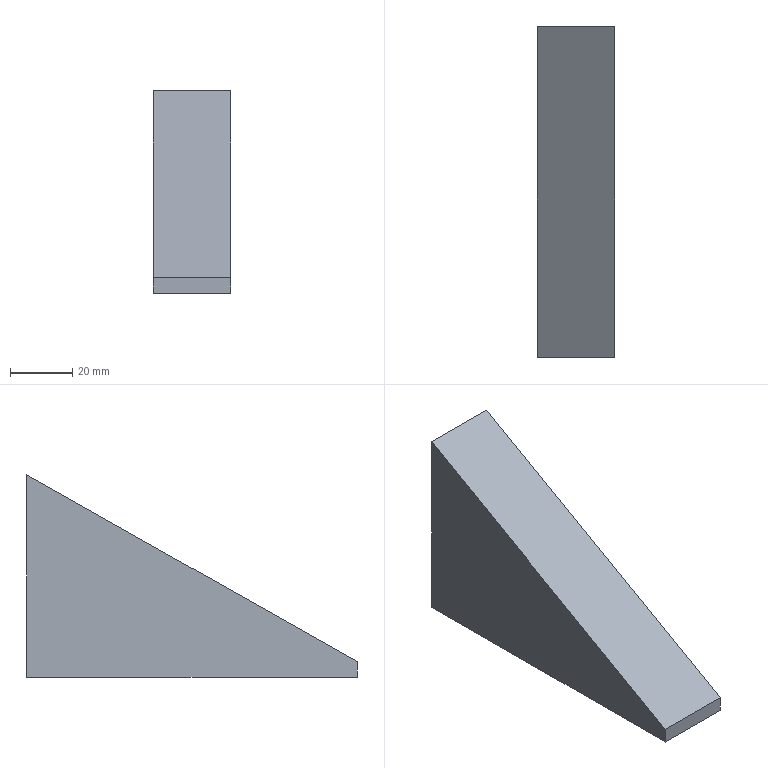Component | SolidWorks | MiddleHousing-1_Stiffener2-1 | 1 solid | 6 faces | box 25 x 106 x 65 mm | volume 92750 mm3 | plane 6
STEP:
#1=COLOUR_RGB('',0.7922,0.8196,0.9333);
#2=FILL_AREA_STYLE_COLOUR('',#1);
#3=FILL_AREA_STYLE('',(#2));
#4=SURFACE_STYLE_FILL_AREA(#3);
#5=SURFACE_SIDE_STYLE('',(#4));
#6=SURFACE_STYLE_USAGE(.BOTH.,#5);
#7=PRESENTATION_STYLE_ASSIGNMENT((#6));
#8=CARTESIAN_POINT('',(4.331,1.181,6.496));
#9=VERTEX_POINT('',#8);
#10=CARTESIAN_POINT('',(4.331,5.354,8.858));
#11=VERTEX_POINT('',#10);
#12=CARTESIAN_POINT('',(4.331,1.181,6.496));
#13=DIRECTION('',(0.,0.8703,0.4926));
#14=VECTOR('',#13,39.37);
#15=LINE('',#12,#14);
#16=EDGE_CURVE('',#9,#11,#15,.T.);
#17=ORIENTED_EDGE('',*,*,#16,.F.);
#18=CARTESIAN_POINT('',(4.331,1.181,6.299));
#19=VERTEX_POINT('',#18);
#20=CARTESIAN_POINT('',(4.331,1.181,8.858));
#21=DIRECTION('',(0.,0.,1.));
#22=VECTOR('',#21,39.37);
#23=LINE('',#20,#22);
#24=EDGE_CURVE('',#19,#9,#23,.T.);
#25=ORIENTED_EDGE('',*,*,#24,.F.);
#26=CARTESIAN_POINT('',(4.331,5.354,6.299));
#27=VERTEX_POINT('',#26);
#28=CARTESIAN_POINT('',(4.331,5.354,6.299));
#29=DIRECTION('',(0.,-1.,0.));
#30=VECTOR('',#29,39.37);
#31=LINE('',#28,#30);
#32=EDGE_CURVE('',#27,#19,#31,.T.);
#33=ORIENTED_EDGE('',*,*,#32,.F.);
#34=CARTESIAN_POINT('',(4.331,5.354,8.858));
#35=DIRECTION('',(0.,0.,-1.));
#36=VECTOR('',#35,39.37);
#37=LINE('',#34,#36);
#38=EDGE_CURVE('',#11,#27,#37,.T.);
#39=ORIENTED_EDGE('',*,*,#38,.F.);
#40=EDGE_LOOP('',(#17,#25,#33,#39));
#41=FACE_OUTER_BOUND('',#40,.T.);
#42=CARTESIAN_POINT('',(4.331,5.354,8.858));
#43=DIRECTION('',(-1.,0.,0.));
#44=DIRECTION('',(0.,0.,1.));
#45=AXIS2_PLACEMENT_3D('',#42,#43,#44);
#46=PLANE('',#45);
#47=ADVANCED_FACE('',(#41),#46,.F.);
#48=CARTESIAN_POINT('',(3.346,5.354,8.858));
#49=VERTEX_POINT('',#48);
#50=CARTESIAN_POINT('',(3.346,5.354,6.299));
#51=VERTEX_POINT('',#50);
#52=CARTESIAN_POINT('',(3.346,5.354,8.858));
#53=DIRECTION('',(0.,0.,-1.));
#54=VECTOR('',#53,39.37);
#55=LINE('',#52,#54);
#56=EDGE_CURVE('',#49,#51,#55,.T.);
#57=ORIENTED_EDGE('',*,*,#56,.F.);
#58=CARTESIAN_POINT('',(3.346,5.354,8.858));
#59=DIRECTION('',(-1.,0.,0.));
#60=VECTOR('',#59,39.37);
#61=LINE('',#58,#60);
#62=EDGE_CURVE('',#11,#49,#61,.T.);
#63=ORIENTED_EDGE('',*,*,#62,.F.);
#64=ORIENTED_EDGE('',*,*,#38,.T.);
#65=CARTESIAN_POINT('',(3.346,5.354,6.299));
#66=DIRECTION('',(1.,0.,0.));
#67=VECTOR('',#66,39.37);
#68=LINE('',#65,#67);
#69=EDGE_CURVE('',#51,#27,#68,.T.);
#70=ORIENTED_EDGE('',*,*,#69,.F.);
#71=EDGE_LOOP('',(#57,#63,#64,#70));
#72=FACE_OUTER_BOUND('',#71,.T.);
#73=CARTESIAN_POINT('',(3.346,5.354,8.858));
#74=DIRECTION('',(0.,-1.,0.));
#75=DIRECTION('',(0.,0.,-1.));
#76=AXIS2_PLACEMENT_3D('',#73,#74,#75);
#77=PLANE('',#76);
#78=ADVANCED_FACE('',(#72),#77,.F.);
#79=CARTESIAN_POINT('',(3.346,1.181,6.496));
#80=VERTEX_POINT('',#79);
#81=CARTESIAN_POINT('',(3.346,1.181,6.496));
#82=DIRECTION('',(0.,0.8703,0.4926));
#83=VECTOR('',#82,39.37);
#84=LINE('',#81,#83);
#85=EDGE_CURVE('',#80,#49,#84,.T.);
#86=ORIENTED_EDGE('',*,*,#85,.F.);
#87=CARTESIAN_POINT('',(20.276,1.181,6.496));
#88=DIRECTION('',(-1.,0.,0.));
#89=VECTOR('',#88,39.37);
#90=LINE('',#87,#89);
#91=EDGE_CURVE('',#9,#80,#90,.T.);
#92=ORIENTED_EDGE('',*,*,#91,.F.);
#93=ORIENTED_EDGE('',*,*,#16,.T.);
#94=ORIENTED_EDGE('',*,*,#62,.T.);
#95=EDGE_LOOP('',(#86,#92,#93,#94));
#96=FACE_OUTER_BOUND('',#95,.T.);
#97=CARTESIAN_POINT('',(20.276,1.181,6.496));
#98=DIRECTION('',(0.,0.4926,-0.8703));
#99=DIRECTION('',(0.,0.8703,0.4926));
#100=AXIS2_PLACEMENT_3D('',#97,#98,#99);
#101=PLANE('',#100);
#102=ADVANCED_FACE('',(#96),#101,.F.);
#103=ORIENTED_EDGE('',*,*,#91,.T.);
#104=CARTESIAN_POINT('',(3.346,1.181,6.299));
#105=VERTEX_POINT('',#104);
#106=CARTESIAN_POINT('',(3.346,1.181,8.858));
#107=DIRECTION('',(0.,0.,1.));
#108=VECTOR('',#107,39.37);
#109=LINE('',#106,#108);
#110=EDGE_CURVE('',#105,#80,#109,.T.);
#111=ORIENTED_EDGE('',*,*,#110,.F.);
#112=CARTESIAN_POINT('',(3.346,1.181,6.299));
#113=DIRECTION('',(-1.,0.,0.));
#114=VECTOR('',#113,39.37);
#115=LINE('',#112,#114);
#116=EDGE_CURVE('',#19,#105,#115,.T.);
#117=ORIENTED_EDGE('',*,*,#116,.F.);
#118=ORIENTED_EDGE('',*,*,#24,.T.);
#119=EDGE_LOOP('',(#103,#111,#117,#118));
#120=FACE_OUTER_BOUND('',#119,.T.);
#121=CARTESIAN_POINT('',(3.346,1.181,8.858));
#122=DIRECTION('',(0.,1.,0.));
#123=DIRECTION('',(0.,0.,1.));
#124=AXIS2_PLACEMENT_3D('',#121,#122,#123);
#125=PLANE('',#124);
#126=ADVANCED_FACE('',(#120),#125,.F.);
#127=ORIENTED_EDGE('',*,*,#69,.T.);
#128=ORIENTED_EDGE('',*,*,#32,.T.);
#129=ORIENTED_EDGE('',*,*,#116,.T.);
#130=CARTESIAN_POINT('',(3.346,0.9843,6.299));
#131=DIRECTION('',(0.,-1.,0.));
#132=VECTOR('',#131,39.37);
#133=LINE('',#130,#132);
#134=EDGE_CURVE('',#51,#105,#133,.T.);
#135=ORIENTED_EDGE('',*,*,#134,.F.);
#136=EDGE_LOOP('',(#127,#128,#129,#135));
#137=FACE_OUTER_BOUND('',#136,.T.);
#138=CARTESIAN_POINT('',(8.268,0.9843,6.299));
#139=DIRECTION('',(0.,0.,1.));
#140=DIRECTION('',(1.,0.,0.));
#141=AXIS2_PLACEMENT_3D('',#138,#139,#140);
#142=PLANE('',#141);
#143=ADVANCED_FACE('',(#137),#142,.F.);
#144=ORIENTED_EDGE('',*,*,#85,.T.);
#145=ORIENTED_EDGE('',*,*,#56,.T.);
#146=ORIENTED_EDGE('',*,*,#134,.T.);
#147=ORIENTED_EDGE('',*,*,#110,.T.);
#148=EDGE_LOOP('',(#144,#145,#146,#147));
#149=FACE_OUTER_BOUND('',#148,.T.);
#150=CARTESIAN_POINT('',(3.346,5.354,8.858));
#151=DIRECTION('',(1.,0.,0.));
#152=DIRECTION('',(0.,0.,-1.));
#153=AXIS2_PLACEMENT_3D('',#150,#151,#152);
#154=PLANE('',#153);
#155=ADVANCED_FACE('',(#149),#154,.F.);
#156=CLOSED_SHELL('',(#47,#78,#102,#126,#143,#155));
#157=MANIFOLD_SOLID_BREP('',#156);
#158=STYLED_ITEM('',(#7),#157);
#159=PRESENTATION_LAYER_ASSIGNMENT('','',(#158));
#160=(LENGTH_UNIT()NAMED_UNIT(*)SI_UNIT($,.METRE.));
#161=LENGTH_MEASURE_WITH_UNIT(LENGTH_MEASURE(0.0254),#160);
#162=DIMENSIONAL_EXPONENTS(1.,0.,0.,0.,0.,0.,0.);
#163=(CONVERSION_BASED_UNIT('',#161)LENGTH_UNIT()NAMED_UNIT(#162));
#164=UNCERTAINTY_MEASURE_WITH_UNIT(LENGTH_MEASURE(0.00001),#163,'','');
#165=(NAMED_UNIT(*)PLANE_ANGLE_UNIT()SI_UNIT($,.RADIAN.));
#166=(NAMED_UNIT(*)SI_UNIT($,.STERADIAN.)SOLID_ANGLE_UNIT());
#167=(GEOMETRIC_REPRESENTATION_CONTEXT(3)GLOBAL_UNCERTAINTY_ASSIGNED_CONTEXT((#164))GLOBAL_UNIT_ASSIGNED_CONTEXT((#163,#165,#166))REPRESENTATION_CONTEXT('',''));
#168=MECHANICAL_DESIGN_GEOMETRIC_PRESENTATION_REPRESENTATION('',(#158),#167);
#169=CARTESIAN_POINT('',(0.,0.,0.));
#170=DIRECTION('',(0.,0.,1.));
#171=DIRECTION('',(1.,0.,0.));
#172=AXIS2_PLACEMENT_3D('',#169,#170,#171);
#173=(LENGTH_UNIT()NAMED_UNIT(*)SI_UNIT($,.METRE.));
#174=LENGTH_MEASURE_WITH_UNIT(LENGTH_MEASURE(0.0254),#173);
#175=DIMENSIONAL_EXPONENTS(1.,0.,0.,0.,0.,0.,0.);
#176=(CONVERSION_BASED_UNIT('',#174)LENGTH_UNIT()NAMED_UNIT(#175));
#177=UNCERTAINTY_MEASURE_WITH_UNIT(LENGTH_MEASURE(0.00001),#176,'','');
#178=(NAMED_UNIT(*)PLANE_ANGLE_UNIT()SI_UNIT($,.RADIAN.));
#179=(NAMED_UNIT(*)SI_UNIT($,.STERADIAN.)SOLID_ANGLE_UNIT());
#180=(GEOMETRIC_REPRESENTATION_CONTEXT(3)GLOBAL_UNCERTAINTY_ASSIGNED_CONTEXT((#177))GLOBAL_UNIT_ASSIGNED_CONTEXT((#176,#178,#179))REPRESENTATION_CONTEXT('',''));
#181=ADVANCED_BREP_SHAPE_REPRESENTATION('',(#157,#172),#180);